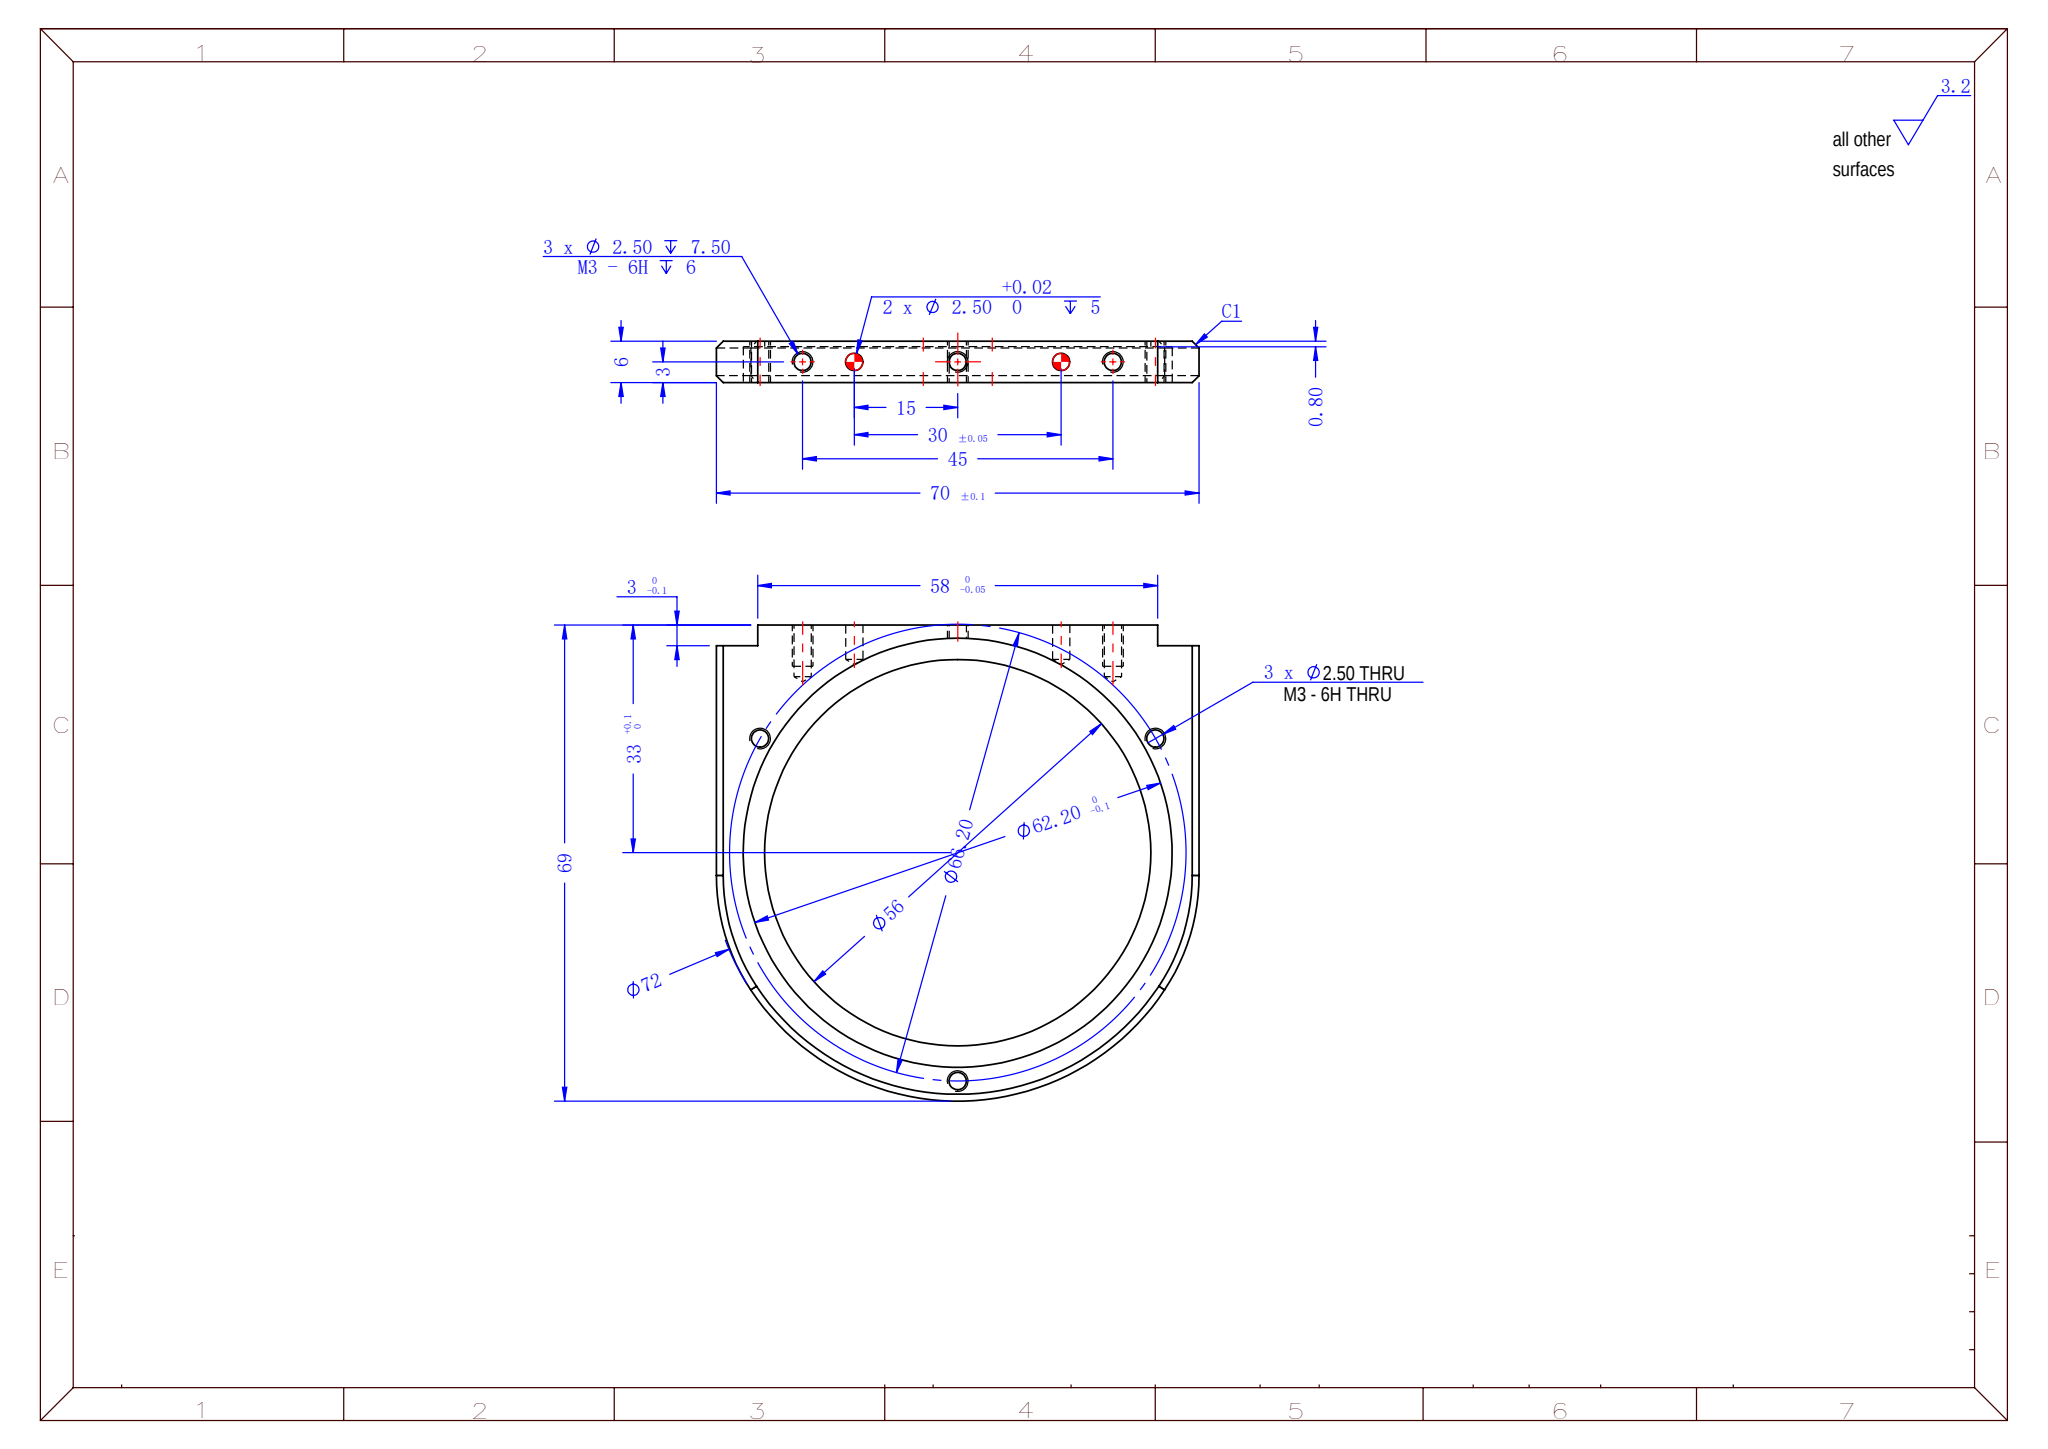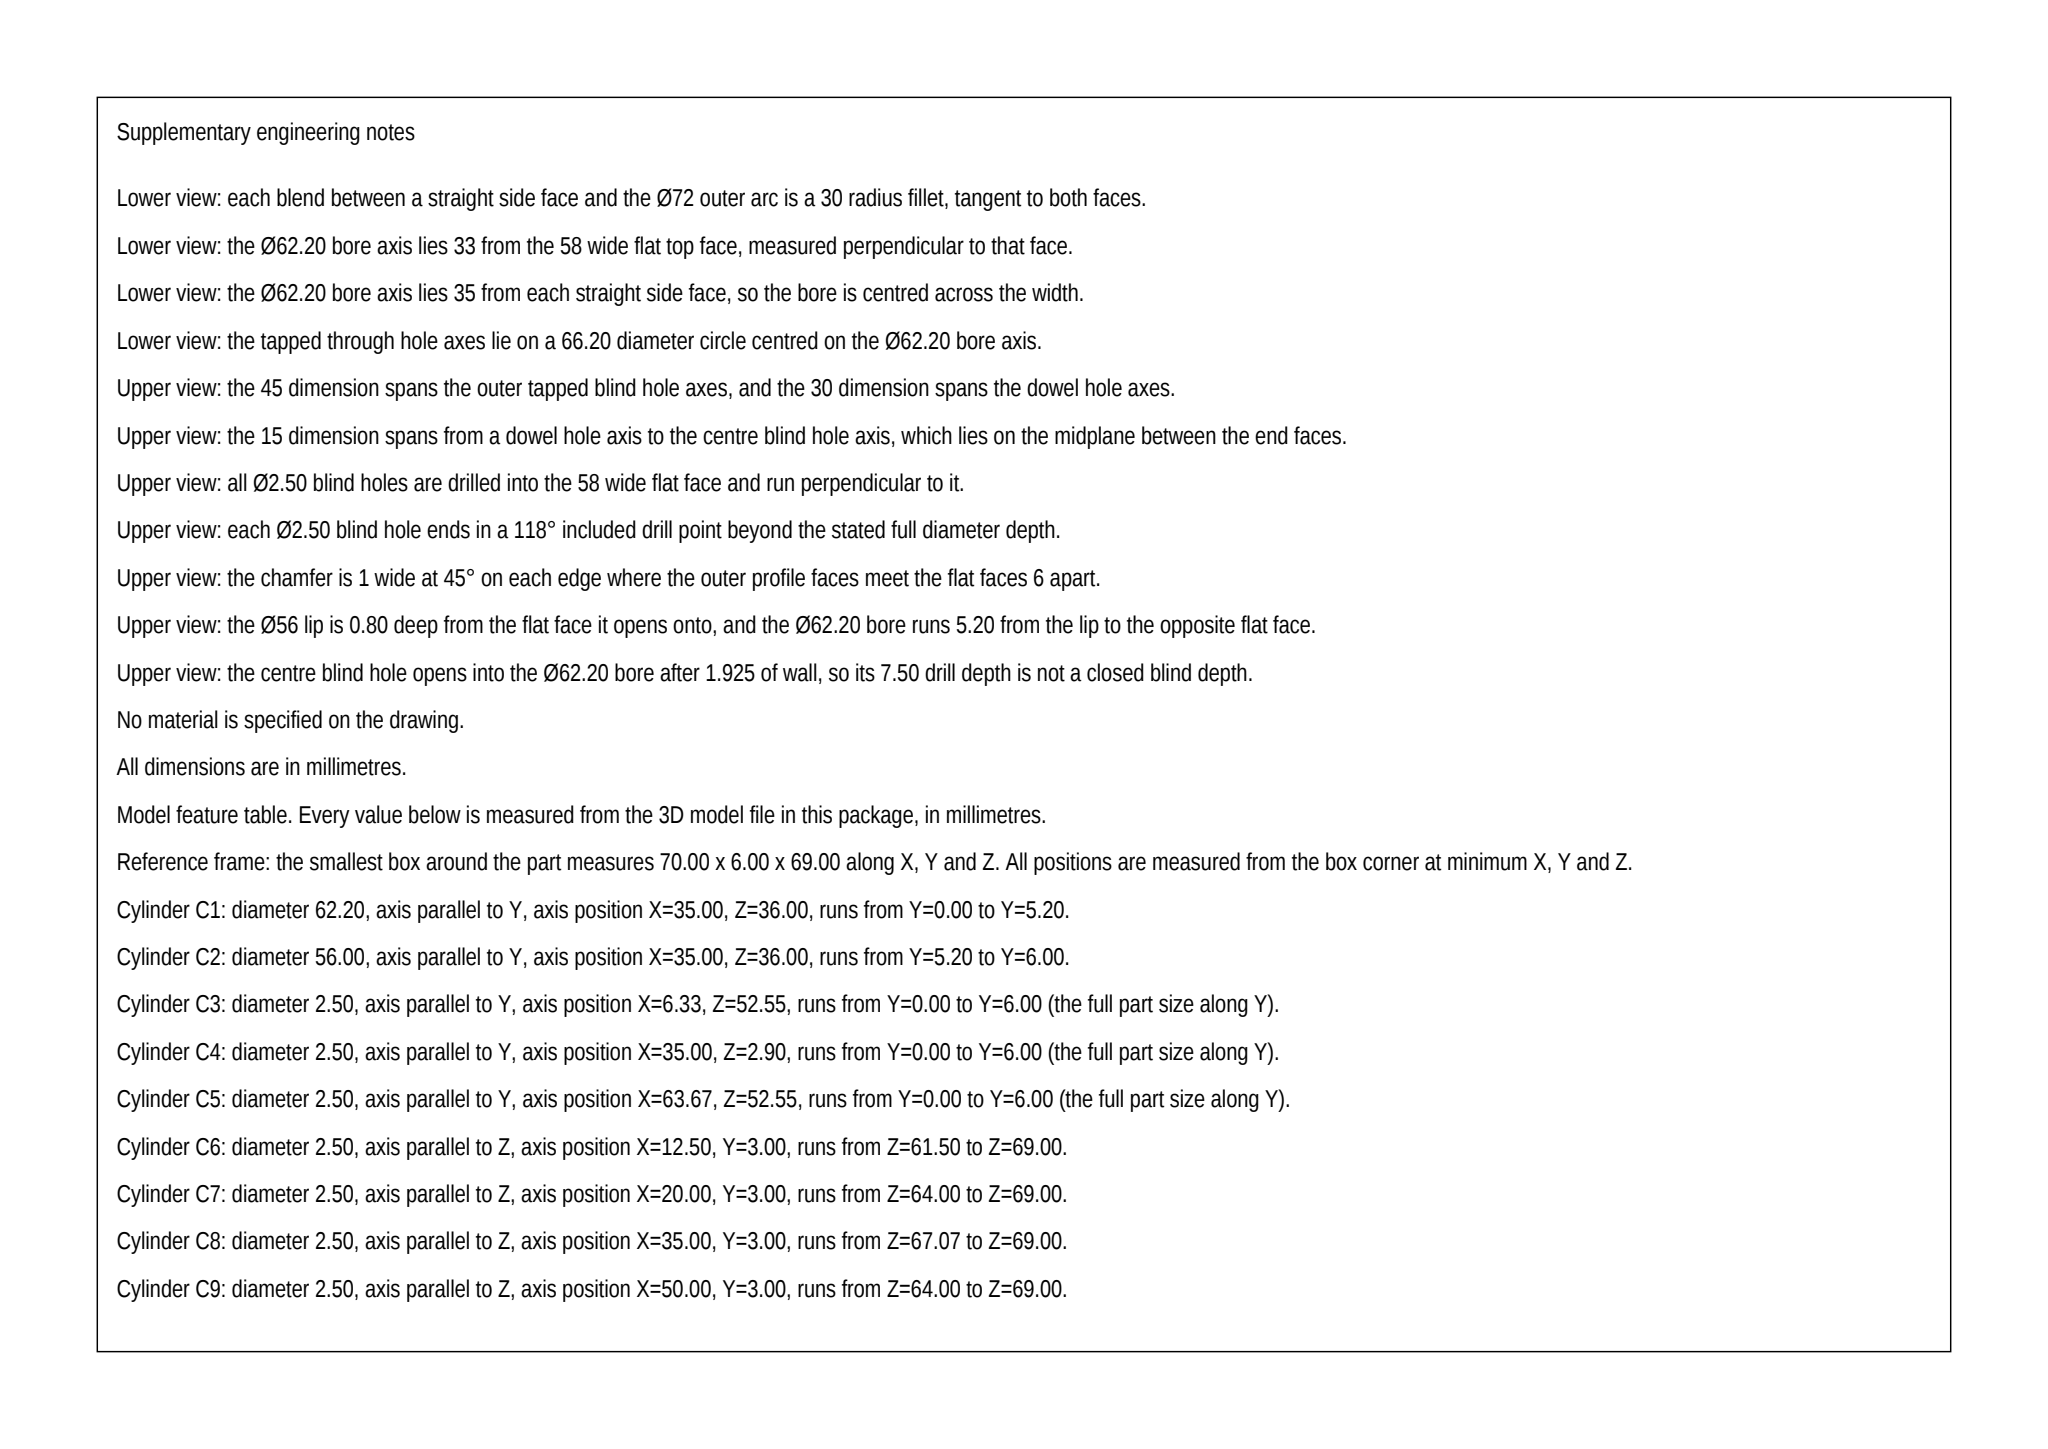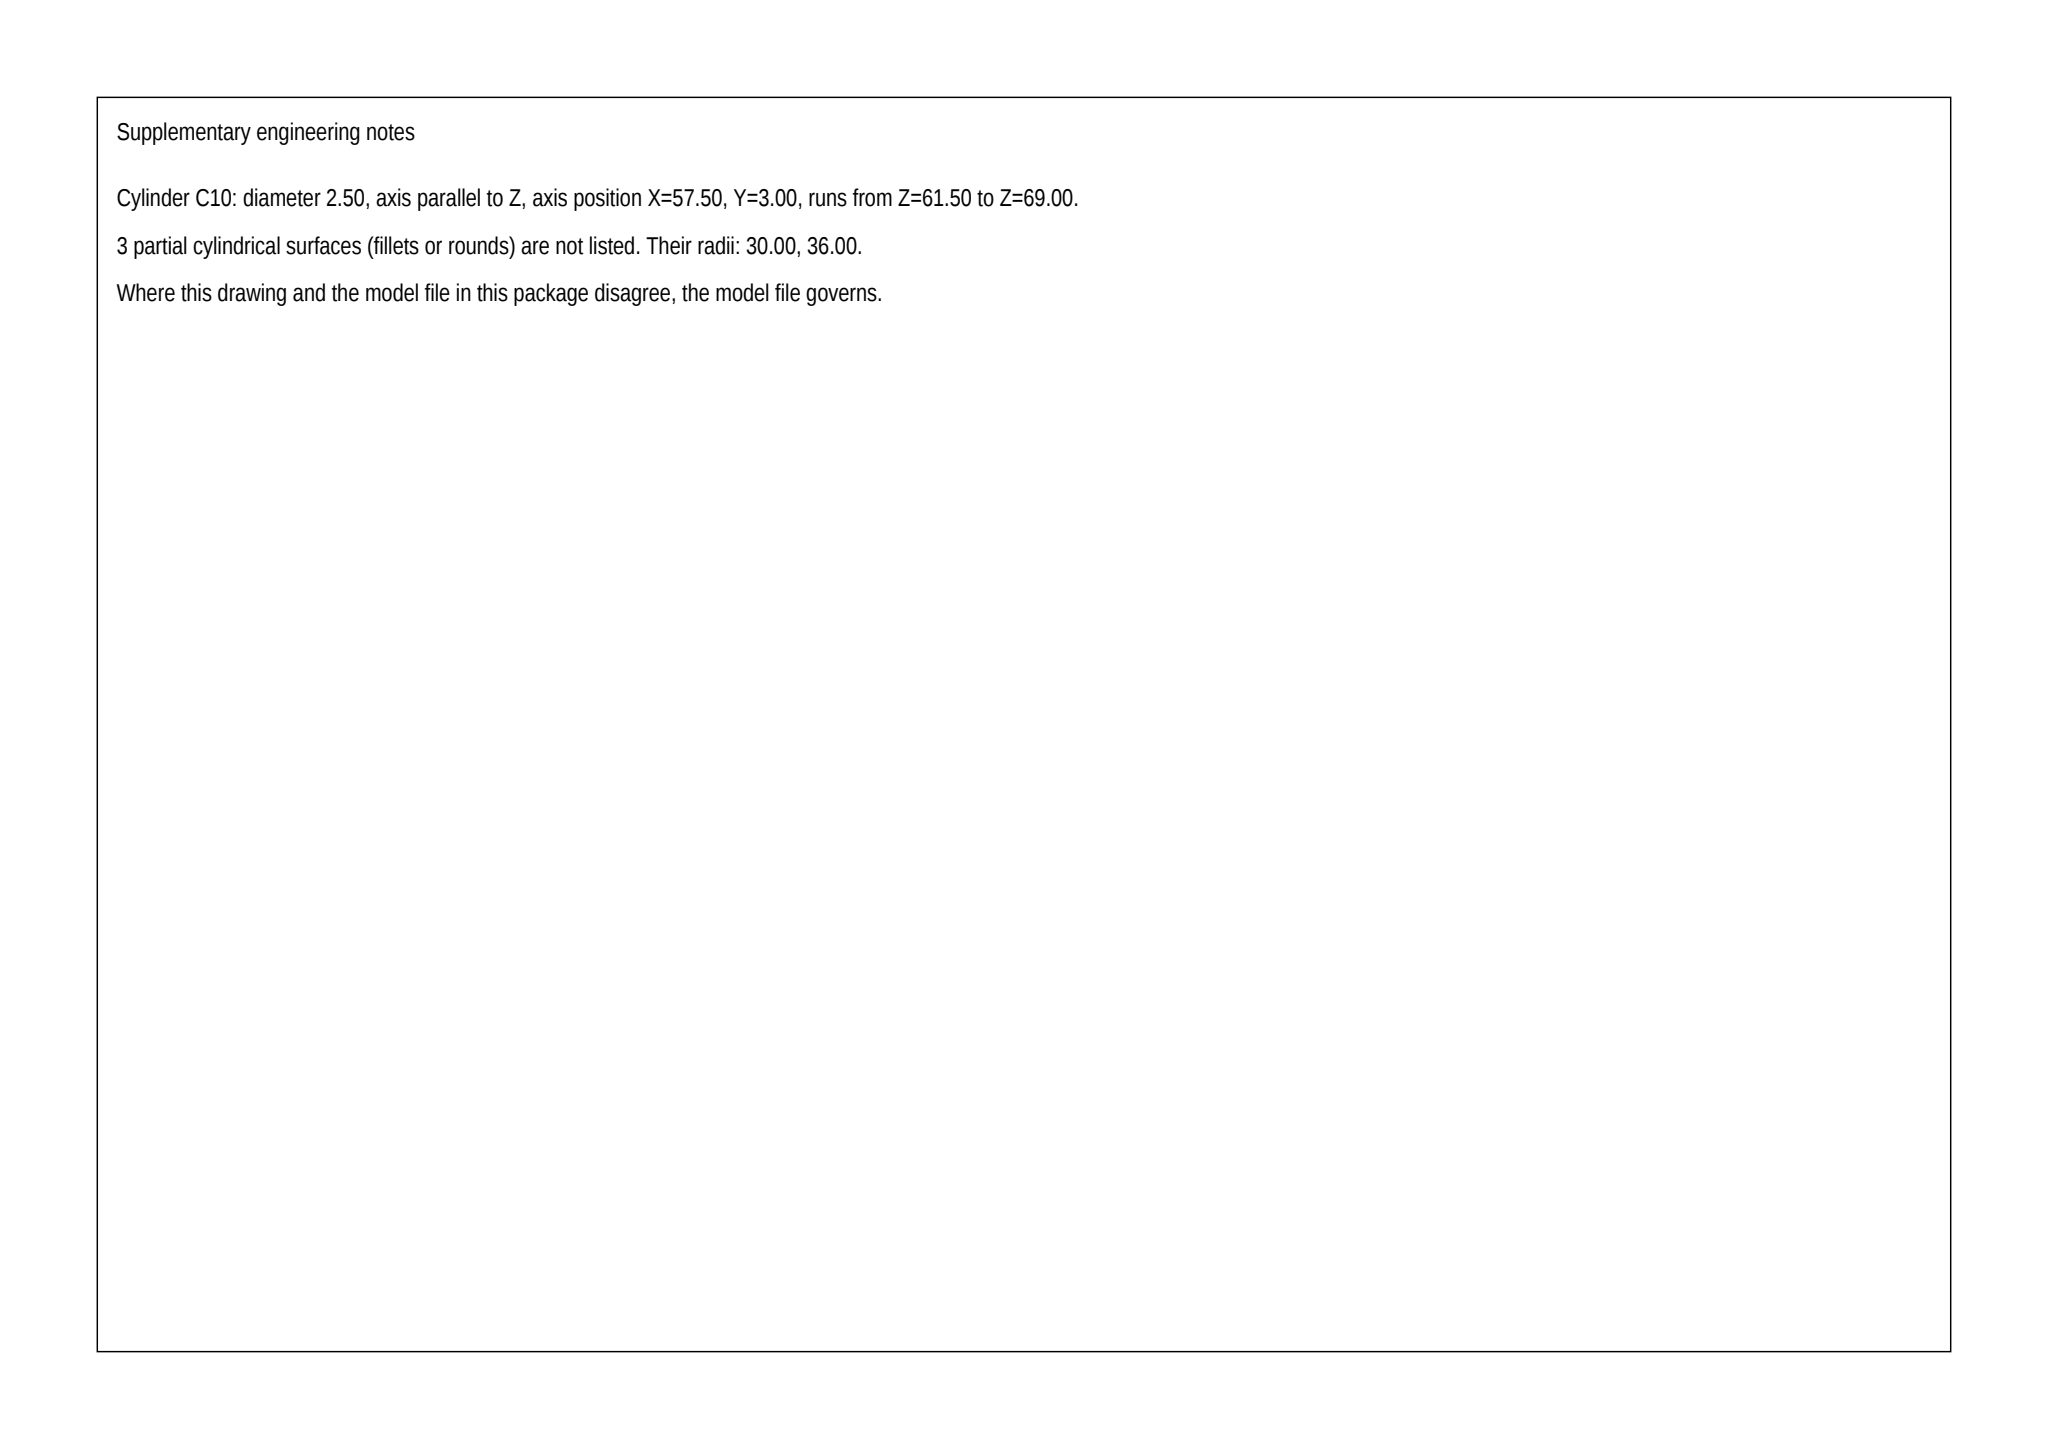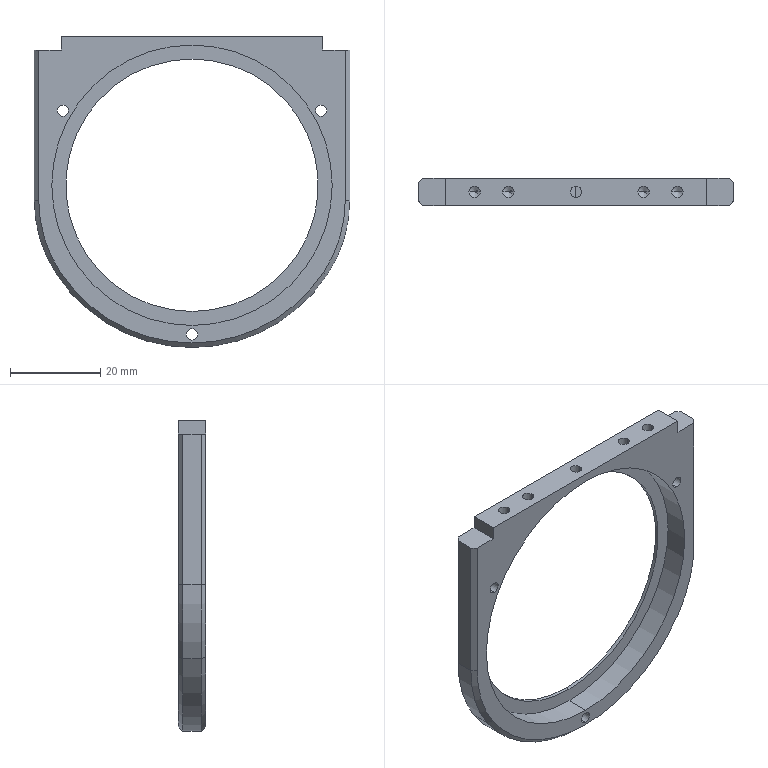Part | SolidWorks | mm | 1 solid | 52 faces | box 70 x 6 x 69 mm | volume 7592 mm3 | cylinder 23 | cone 15 | plane 14 | commonest cylinder face diameters 2.5 x16 62.2 x2 56 x2 60 x2 72 x1
build123d program:
from build123d import *

# Parameters (mm, degrees)
SKETCH1_W                     = 70
SKETCH1_H                     = 70
BOSS_EXTRUDE1_DEPTH           = 3
SKETCH2_OUTSIDE_W             = 91.836
SKETCH2_OUTSIDE_H             = 27.836
SKETCH2_OUTSIDE_W_2           = 58
SKETCH2_OUTSIDE_H_2           = 6
CUT_EXTRUDE1_DEPTH            = 3
M3_TAPPED_HOLE1_D             = 2.5
M3_TAPPED_HOLE1_DEPTH         = 7.5
M3_TAPPED_HOLE1_TIP           = 0.7511
SIZE_MM_DOWEL_PIN_HOLE1_D     = 2.5
SIZE_MM_DOWEL_PIN_HOLE1_DEPTH = 5
SIZE_MM_DOWEL_PIN_HOLE1_TIP   = 0.7511
CUT_EXTRUDE2_REACH            = 51.86
SKETCH7_R                     = 28
SKETCH8_R                     = 31.1
CUT_EXTRUDE3_DEPTH            = 5.2
M3_TAPPED_HOLE2_D             = 2.5
CIRPATTERN1_COUNT             = 3
FILLET1_R                     = 30
CHAMFER1_SIZE                 = 1


with BuildPart() as part:
    # Sketch1 → Boss-Extrude1 (new, symmetric)
    with BuildSketch(Plane(origin=(0, 0, 0), x_dir=(1, 0, 0), z_dir=(0, 1, 0))):
        Rectangle(SKETCH1_W, SKETCH1_H)
    extrude(amount=BOSS_EXTRUDE1_DEPTH, both=True)

    # Sketch2 outside → Cut-Extrude1 (cut)
    with BuildSketch(Plane.XY.offset(35)):
        Rectangle(SKETCH2_OUTSIDE_W, SKETCH2_OUTSIDE_H)
        Rectangle(SKETCH2_OUTSIDE_W_2, SKETCH2_OUTSIDE_H_2, mode=Mode.SUBTRACT)
    extrude(amount=-CUT_EXTRUDE1_DEPTH, mode=Mode.SUBTRACT)

    # M3 Tapped Hole1
    with Locations(Plane.XY.offset(35)):
        with Locations((-22.5, 0), (22.5, 0), (0, 0)):
            Hole(M3_TAPPED_HOLE1_D / 2, depth=M3_TAPPED_HOLE1_DEPTH)
            with Locations((0, 0, -(M3_TAPPED_HOLE1_DEPTH + M3_TAPPED_HOLE1_TIP / 2))):  # 118° drill point
                Cone(0, M3_TAPPED_HOLE1_D / 2, M3_TAPPED_HOLE1_TIP, mode=Mode.SUBTRACT)

    # Size mm Dowel Pin Hole1
    with Locations(Plane.XY.offset(35)):
        with Locations((-15, 0), (15, 0)):
            Hole(SIZE_MM_DOWEL_PIN_HOLE1_D / 2, depth=SIZE_MM_DOWEL_PIN_HOLE1_DEPTH)
            with Locations((0, 0, -(SIZE_MM_DOWEL_PIN_HOLE1_DEPTH + SIZE_MM_DOWEL_PIN_HOLE1_TIP / 2))):  # 118° drill point
                Cone(0, SIZE_MM_DOWEL_PIN_HOLE1_D / 2, SIZE_MM_DOWEL_PIN_HOLE1_TIP, mode=Mode.SUBTRACT)

    # Sketch7 → Cut-Extrude2 (cut, up to next)
    with BuildSketch(Plane(origin=(0, 3, 0), x_dir=(1, 0, 0), z_dir=(0, 1, 0)), mode=Mode.PRIVATE) as cut_extrude2_sk1:
        with Locations(Location((0, -2, 0), (0, 0, 270))):
            Circle(SKETCH7_R)
    cut_extrude2_tool1 = extrude(cut_extrude2_sk1.sketch, amount=-CUT_EXTRUDE2_REACH, mode=Mode.PRIVATE) & part.part
    # Sketch7 → Cut-Extrude2 (cut, up to next)
    with BuildSketch(Plane(origin=(0, 3, 0), x_dir=(1, 0, 0), z_dir=(0, 1, 0)), mode=Mode.PRIVATE) as cut_extrude2_sk2:
        with BuildLine():
            Line((-35, 35), (35, 35))
            Line((35, 35), (35, 6.426))
            ThreePointArc((35, 6.426), (0, 34), (-35, 6.426))
            Line((-35, 6.426), (-35, 35))
        make_face()
    cut_extrude2_tool2 = extrude(cut_extrude2_sk2.sketch, amount=-CUT_EXTRUDE2_REACH, mode=Mode.PRIVATE) & part.part
    add(cut_extrude2_tool1.solids().sort_by_distance((0, 3, 2))[0], mode=Mode.SUBTRACT)
    add(cut_extrude2_tool2.solids().sort_by_distance((-34.244, 3, -20.713))[0], mode=Mode.SUBTRACT)

    # Sketch8 → Cut-Extrude3 (cut)
    with BuildSketch(Plane(origin=(0, -3, 0), x_dir=(1, 0, 0), z_dir=(0, 1, 0))):
        with Locations(Location((0, -2, 0), (0, 0, 270))):
            Circle(SKETCH8_R)
    extrude(amount=CUT_EXTRUDE3_DEPTH, mode=Mode.SUBTRACT)

    # M3 Tapped Hole2 (through all)
    with Locations(Plane(origin=(0, -3, 0), x_dir=(-1, 0, 0), z_dir=(0, -1, 0))):
        with Locations((0, 31.1)):
            m3_tapped_hole2 = Hole(M3_TAPPED_HOLE2_D / 2)

    # CirPattern1: M3 Tapped Hole2 ×3 about axis
    cirpattern1_axis = Axis((0, 0, 2), (0, 1, 0))
    for i in range(1, CIRPATTERN1_COUNT):
        add(m3_tapped_hole2.rotate(cirpattern1_axis, i * 360 / CIRPATTERN1_COUNT), mode=Mode.SUBTRACT)

    # Fillet1
    fillet1_edges = [part.edges().sort_by_distance(p)[0] for p in [
        (35, 0, -6.426),
        (-35, 0, -6.426),
    ]]
    fillet(fillet1_edges, radius=FILLET1_R)

    # Chamfer1
    chamfer1_edges = [part.edges().sort_by_distance(p)[0] for p in [
        (0, -3, -34),
        (0, 3, -34),
        (-35, 3, 15.342),
        (33.723, 3, -9.977),
        (-33.723, 3, -9.977),
        (-35, -3, 15.342),
        (33.723, -3, -9.977),
        (-33.723, -3, -9.977),
        (35, -3, 15.342),
        (35, 3, 15.342),
    ]]
    chamfer(chamfer1_edges, length=CHAMFER1_SIZE)


solid = part.part